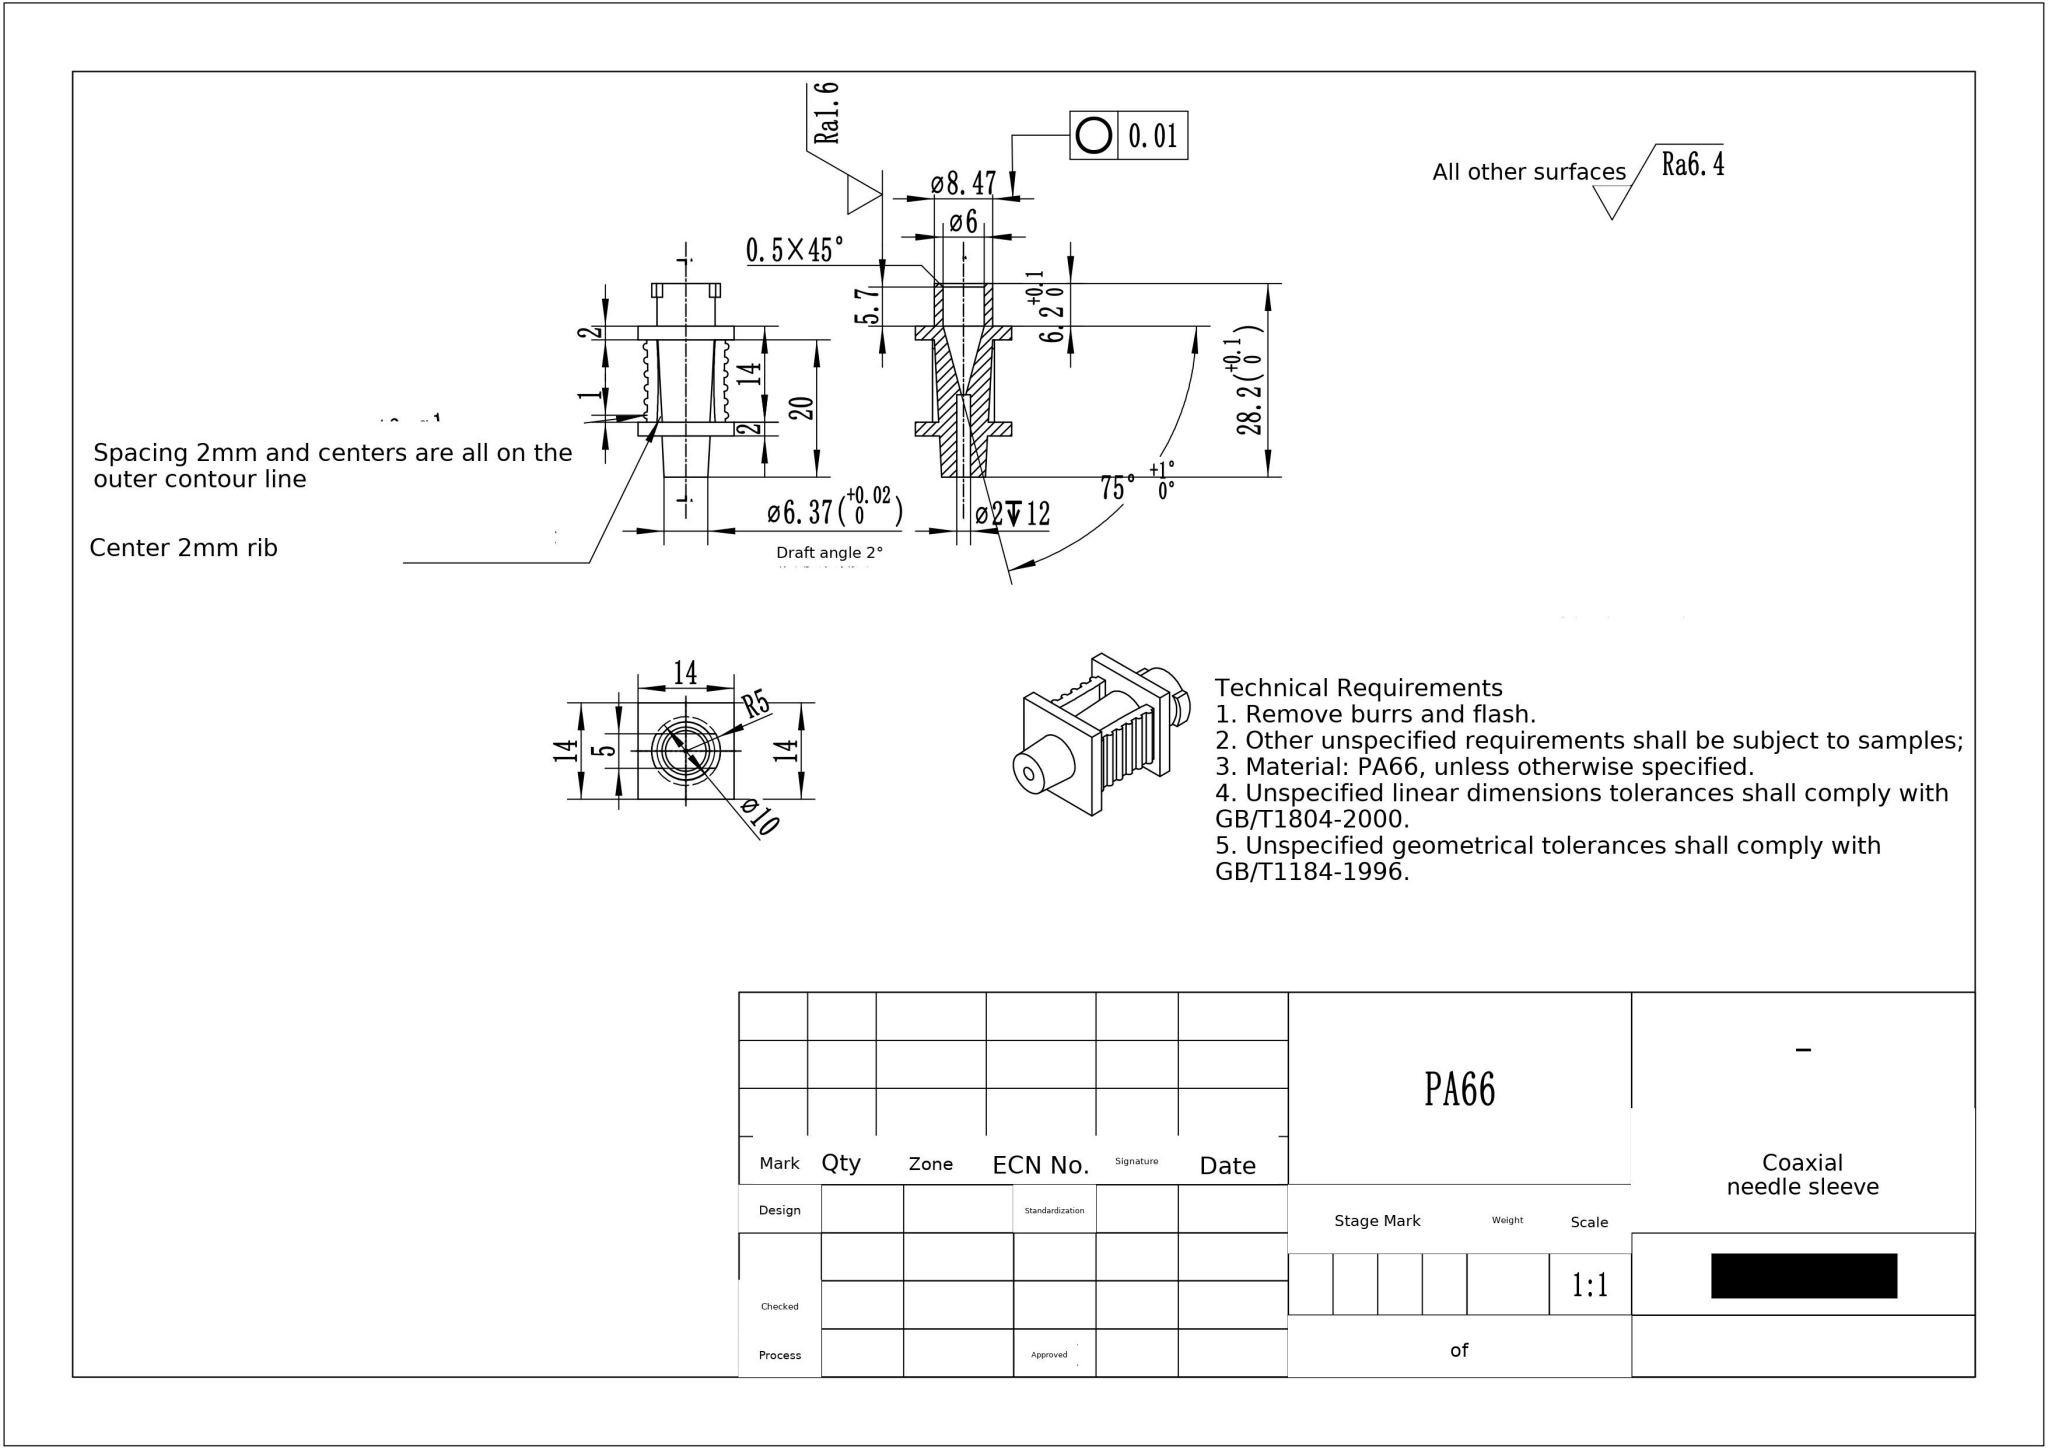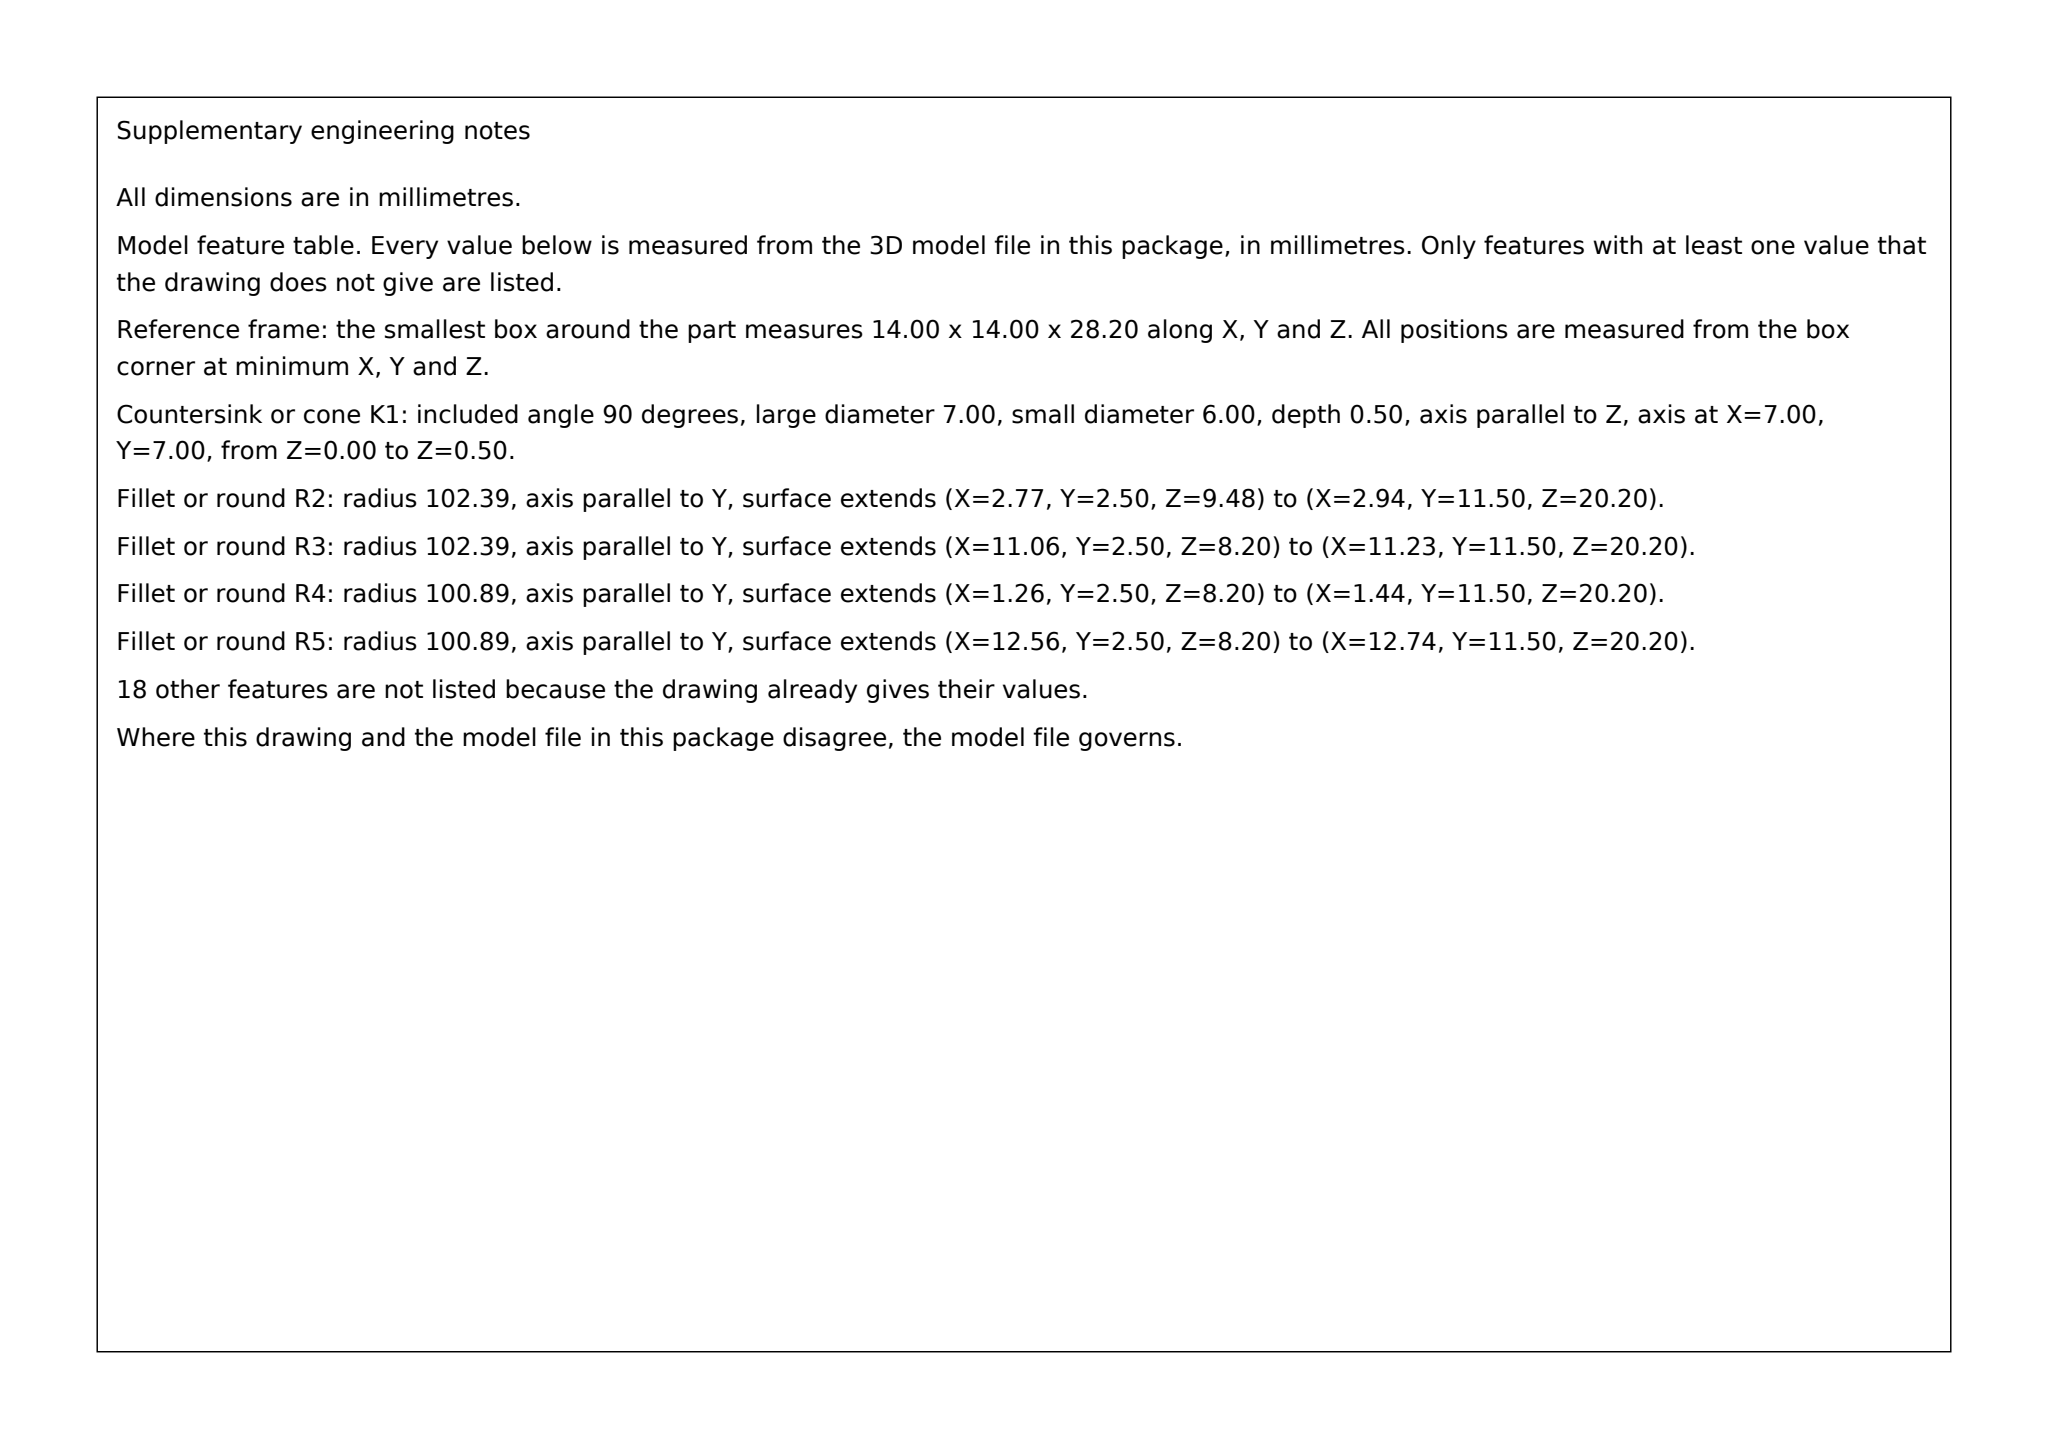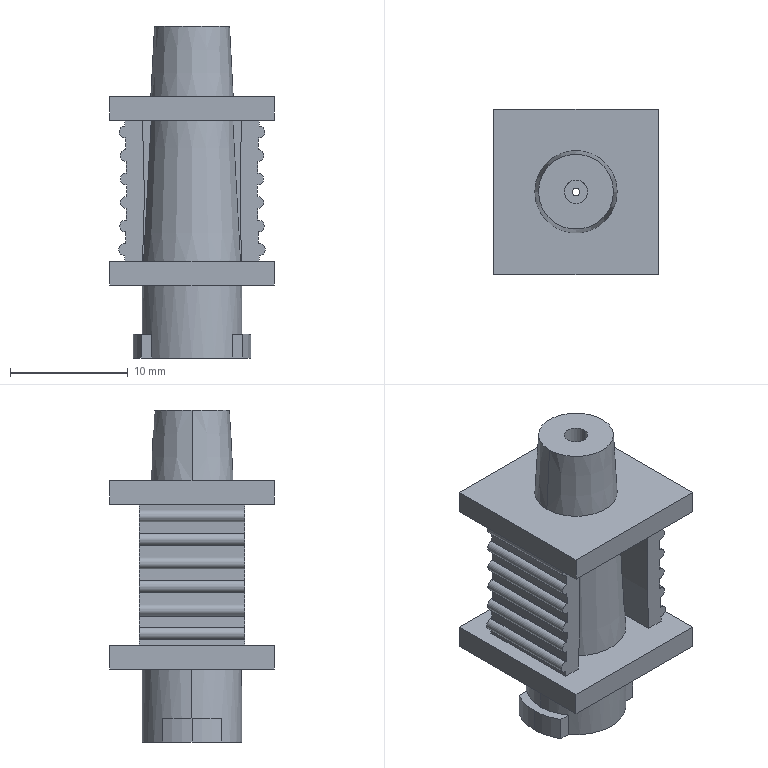Part | SolidWorks | mm | material PA66 | 1 solid | 94 faces | box 14 x 14 x 28.2 mm | volume 2000 mm3 | cylinder 55 | plane 31 | cone 8 | commonest cylinder face diameters 1 x28 201.786 x14 204.786 x4 10 x3 6 x2 8.47 x2 2 x2